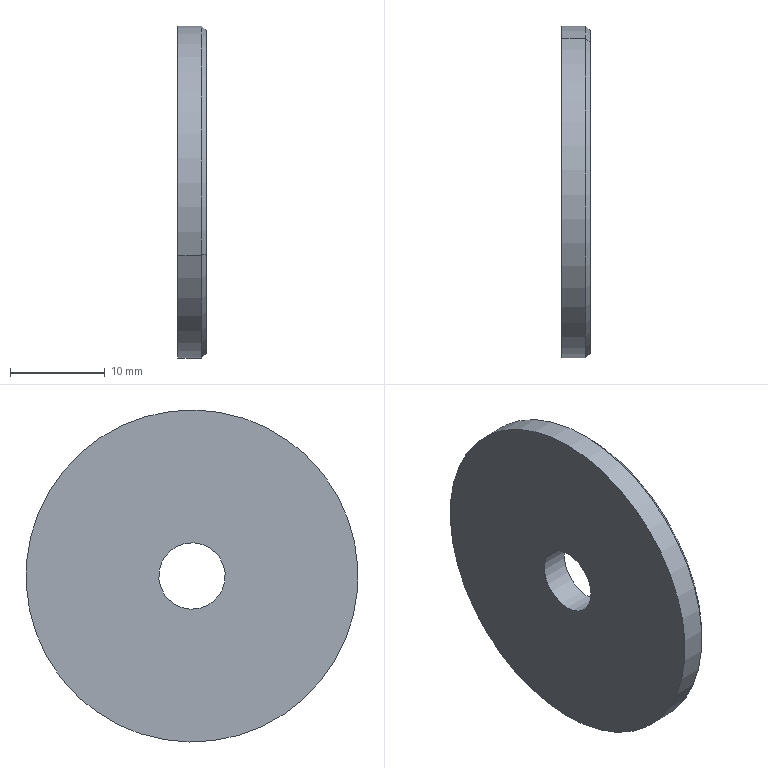Component | SolidWorks | DoubleFilmTransport-1_AxisEndCap-2 | 1 solid | 8 faces | box 3 x 35 x 35 mm | volume 2757 mm3 | cylinder 4 | cone 2 | plane 2 | commonest cylinder face diameters 35 x2 7 x2
build123d program:
from build123d import *


with BuildPart() as part:
    # Sketch1 → Revolve1 (revolve)
    with BuildSketch(Plane(origin=(0, 0, 0), x_dir=(1, 0, 0), z_dir=(0, 1, 0))):
        Polygon((3.5, -3), (17, -3), (17.5, -2.5), (17.5, 0), (3.5, 0), align=None)
    revolve(axis=Axis((0, 0, 0), (0, 0, 1)))


solid = part.part

# Placed as in the assembly
solid = solid.moved(Location((-468.246, 45.373, 13.5), (0, 90, 0)))
STEP:
#1=COLOUR_RGB('',0.7922,0.8196,0.9333);
#2=FILL_AREA_STYLE_COLOUR('',#1);
#3=FILL_AREA_STYLE('',(#2));
#4=SURFACE_STYLE_FILL_AREA(#3);
#5=SURFACE_SIDE_STYLE('',(#4));
#6=SURFACE_STYLE_USAGE(.BOTH.,#5);
#7=PRESENTATION_STYLE_ASSIGNMENT((#6));
#8=CARTESIAN_POINT('',(-18.435,1.15,0.2684));
#9=VERTEX_POINT('',#8);
#10=CARTESIAN_POINT('',(-18.435,2.423,0.7946));
#11=VERTEX_POINT('',#10);
#12=CARTESIAN_POINT('',(-18.435,1.786,0.5315));
#13=DIRECTION('',(1.,0.,0.));
#14=DIRECTION('',(0.,-0.9242,-0.3818));
#15=AXIS2_PLACEMENT_3D('',#12,#13,#14);
#16=CIRCLE('',#15,0.689);
#17=EDGE_CURVE('',#9,#11,#16,.T.);
#18=ORIENTED_EDGE('',*,*,#17,.T.);
#19=CARTESIAN_POINT('',(-18.336,2.423,0.7946));
#20=VERTEX_POINT('',#19);
#21=CARTESIAN_POINT('',(-18.435,2.423,0.7946));
#22=DIRECTION('',(1.,0.,0.));
#23=VECTOR('',#22,39.37);
#24=LINE('',#21,#23);
#25=EDGE_CURVE('',#11,#20,#24,.T.);
#26=ORIENTED_EDGE('',*,*,#25,.T.);
#27=CARTESIAN_POINT('',(-18.336,1.15,0.2684));
#28=VERTEX_POINT('',#27);
#29=CARTESIAN_POINT('',(-18.336,1.786,0.5315));
#30=DIRECTION('',(1.,0.,0.));
#31=DIRECTION('',(0.,-0.9242,-0.3818));
#32=AXIS2_PLACEMENT_3D('',#29,#30,#31);
#33=CIRCLE('',#32,0.689);
#34=EDGE_CURVE('',#28,#20,#33,.T.);
#35=ORIENTED_EDGE('',*,*,#34,.F.);
#36=CARTESIAN_POINT('',(-18.435,1.15,0.2684));
#37=DIRECTION('',(1.,0.,0.));
#38=VECTOR('',#37,39.37);
#39=LINE('',#36,#38);
#40=EDGE_CURVE('',#9,#28,#39,.T.);
#41=ORIENTED_EDGE('',*,*,#40,.F.);
#42=EDGE_LOOP('',(#18,#26,#35,#41));
#43=FACE_OUTER_BOUND('',#42,.T.);
#44=CARTESIAN_POINT('',(-18.435,1.786,0.5315));
#45=DIRECTION('',(1.,0.,0.));
#46=DIRECTION('',(0.,-0.9242,-0.3818));
#47=AXIS2_PLACEMENT_3D('',#44,#45,#46);
#48=CYLINDRICAL_SURFACE('',#47,0.689);
#49=ADVANCED_FACE('',(#43),#48,.T.);
#50=CARTESIAN_POINT('',(-18.317,1.168,0.2759));
#51=VERTEX_POINT('',#50);
#52=CARTESIAN_POINT('',(-18.317,2.405,0.7871));
#53=VERTEX_POINT('',#52);
#54=CARTESIAN_POINT('',(-18.317,1.786,0.5315));
#55=DIRECTION('',(1.,0.,0.));
#56=DIRECTION('',(0.,-0.9242,-0.3818));
#57=AXIS2_PLACEMENT_3D('',#54,#55,#56);
#58=CIRCLE('',#57,0.6693);
#59=EDGE_CURVE('',#51,#53,#58,.T.);
#60=ORIENTED_EDGE('',*,*,#59,.F.);
#61=CARTESIAN_POINT('',(-18.317,1.168,0.2759));
#62=DIRECTION('',(-0.7071,-0.6535,-0.27));
#63=VECTOR('',#62,39.37);
#64=LINE('',#61,#63);
#65=EDGE_CURVE('',#51,#28,#64,.T.);
#66=ORIENTED_EDGE('',*,*,#65,.T.);
#67=ORIENTED_EDGE('',*,*,#34,.T.);
#68=CARTESIAN_POINT('',(-18.317,2.405,0.7871));
#69=DIRECTION('',(-0.7071,0.6535,0.27));
#70=VECTOR('',#69,39.37);
#71=LINE('',#68,#70);
#72=EDGE_CURVE('',#53,#20,#71,.T.);
#73=ORIENTED_EDGE('',*,*,#72,.F.);
#74=EDGE_LOOP('',(#60,#66,#67,#73));
#75=FACE_OUTER_BOUND('',#74,.T.);
#76=CARTESIAN_POINT('',(-18.317,1.786,0.5315));
#77=DIRECTION('',(-1.,-0.,-0.));
#78=DIRECTION('',(0.,0.9242,0.3818));
#79=AXIS2_PLACEMENT_3D('',#76,#77,#78);
#80=CONICAL_SURFACE('',#79,0.6693,0.7854);
#81=ADVANCED_FACE('',(#75),#80,.T.);
#82=CARTESIAN_POINT('',(-18.435,1.914,0.5841));
#83=VERTEX_POINT('',#82);
#84=CARTESIAN_POINT('',(-18.435,1.659,0.4789));
#85=VERTEX_POINT('',#84);
#86=CARTESIAN_POINT('',(-18.435,1.786,0.5315));
#87=DIRECTION('',(1.,0.,0.));
#88=DIRECTION('',(0.,-0.9242,-0.3818));
#89=AXIS2_PLACEMENT_3D('',#86,#87,#88);
#90=CIRCLE('',#89,0.1378);
#91=EDGE_CURVE('',#83,#85,#90,.T.);
#92=ORIENTED_EDGE('',*,*,#91,.F.);
#93=CARTESIAN_POINT('',(-18.317,1.914,0.5841));
#94=VERTEX_POINT('',#93);
#95=CARTESIAN_POINT('',(-18.435,1.914,0.5841));
#96=DIRECTION('',(1.,0.,0.));
#97=VECTOR('',#96,39.37);
#98=LINE('',#95,#97);
#99=EDGE_CURVE('',#83,#94,#98,.T.);
#100=ORIENTED_EDGE('',*,*,#99,.T.);
#101=CARTESIAN_POINT('',(-18.317,1.659,0.4789));
#102=VERTEX_POINT('',#101);
#103=CARTESIAN_POINT('',(-18.317,1.786,0.5315));
#104=DIRECTION('',(1.,0.,0.));
#105=DIRECTION('',(0.,-0.9242,-0.3818));
#106=AXIS2_PLACEMENT_3D('',#103,#104,#105);
#107=CIRCLE('',#106,0.1378);
#108=EDGE_CURVE('',#94,#102,#107,.T.);
#109=ORIENTED_EDGE('',*,*,#108,.T.);
#110=CARTESIAN_POINT('',(-18.435,1.659,0.4789));
#111=DIRECTION('',(1.,0.,0.));
#112=VECTOR('',#111,39.37);
#113=LINE('',#110,#112);
#114=EDGE_CURVE('',#85,#102,#113,.T.);
#115=ORIENTED_EDGE('',*,*,#114,.F.);
#116=EDGE_LOOP('',(#92,#100,#109,#115));
#117=FACE_OUTER_BOUND('',#116,.T.);
#118=CARTESIAN_POINT('',(-18.435,1.786,0.5315));
#119=DIRECTION('',(1.,0.,0.));
#120=DIRECTION('',(0.,-0.9242,-0.3818));
#121=AXIS2_PLACEMENT_3D('',#118,#119,#120);
#122=CYLINDRICAL_SURFACE('',#121,0.1378);
#123=ADVANCED_FACE('',(#117),#122,.F.);
#124=ORIENTED_EDGE('',*,*,#99,.F.);
#125=CARTESIAN_POINT('',(-18.435,1.786,0.5315));
#126=DIRECTION('',(1.,0.,0.));
#127=DIRECTION('',(0.,-0.9242,-0.3818));
#128=AXIS2_PLACEMENT_3D('',#125,#126,#127);
#129=CIRCLE('',#128,0.1378);
#130=EDGE_CURVE('',#85,#83,#129,.T.);
#131=ORIENTED_EDGE('',*,*,#130,.F.);
#132=ORIENTED_EDGE('',*,*,#114,.T.);
#133=CARTESIAN_POINT('',(-18.317,1.786,0.5315));
#134=DIRECTION('',(1.,0.,0.));
#135=DIRECTION('',(0.,-0.9242,-0.3818));
#136=AXIS2_PLACEMENT_3D('',#133,#134,#135);
#137=CIRCLE('',#136,0.1378);
#138=EDGE_CURVE('',#102,#94,#137,.T.);
#139=ORIENTED_EDGE('',*,*,#138,.T.);
#140=EDGE_LOOP('',(#124,#131,#132,#139));
#141=FACE_OUTER_BOUND('',#140,.T.);
#142=CARTESIAN_POINT('',(-18.435,1.786,0.5315));
#143=DIRECTION('',(1.,0.,0.));
#144=DIRECTION('',(0.,-0.9242,-0.3818));
#145=AXIS2_PLACEMENT_3D('',#142,#143,#144);
#146=CYLINDRICAL_SURFACE('',#145,0.1378);
#147=ADVANCED_FACE('',(#141),#146,.F.);
#148=CARTESIAN_POINT('',(-18.317,1.786,0.5315));
#149=DIRECTION('',(1.,0.,0.));
#150=DIRECTION('',(0.,-0.9242,-0.3818));
#151=AXIS2_PLACEMENT_3D('',#148,#149,#150);
#152=CIRCLE('',#151,0.6693);
#153=EDGE_CURVE('',#53,#51,#152,.T.);
#154=ORIENTED_EDGE('',*,*,#153,.T.);
#155=ORIENTED_EDGE('',*,*,#59,.T.);
#156=EDGE_LOOP('',(#154,#155));
#157=FACE_OUTER_BOUND('',#156,.T.);
#158=ORIENTED_EDGE('',*,*,#138,.F.);
#159=ORIENTED_EDGE('',*,*,#108,.F.);
#160=EDGE_LOOP('',(#158,#159));
#161=FACE_BOUND('',#160,.T.);
#162=CARTESIAN_POINT('',(-18.317,1.659,0.4789));
#163=DIRECTION('',(1.,0.,0.));
#164=DIRECTION('',(0.,-0.9242,-0.3818));
#165=AXIS2_PLACEMENT_3D('',#162,#163,#164);
#166=PLANE('',#165);
#167=ADVANCED_FACE('',(#157,#161),#166,.T.);
#168=ORIENTED_EDGE('',*,*,#65,.F.);
#169=ORIENTED_EDGE('',*,*,#153,.F.);
#170=ORIENTED_EDGE('',*,*,#72,.T.);
#171=CARTESIAN_POINT('',(-18.336,1.786,0.5315));
#172=DIRECTION('',(1.,0.,0.));
#173=DIRECTION('',(0.,-0.9242,-0.3818));
#174=AXIS2_PLACEMENT_3D('',#171,#172,#173);
#175=CIRCLE('',#174,0.689);
#176=EDGE_CURVE('',#20,#28,#175,.T.);
#177=ORIENTED_EDGE('',*,*,#176,.T.);
#178=EDGE_LOOP('',(#168,#169,#170,#177));
#179=FACE_OUTER_BOUND('',#178,.T.);
#180=CARTESIAN_POINT('',(-18.317,1.786,0.5315));
#181=DIRECTION('',(-1.,-0.,-0.));
#182=DIRECTION('',(0.,0.9242,0.3818));
#183=AXIS2_PLACEMENT_3D('',#180,#181,#182);
#184=CONICAL_SURFACE('',#183,0.6693,0.7854);
#185=ADVANCED_FACE('',(#179),#184,.T.);
#186=ORIENTED_EDGE('',*,*,#25,.F.);
#187=CARTESIAN_POINT('',(-18.435,1.786,0.5315));
#188=DIRECTION('',(1.,0.,0.));
#189=DIRECTION('',(0.,-0.9242,-0.3818));
#190=AXIS2_PLACEMENT_3D('',#187,#188,#189);
#191=CIRCLE('',#190,0.689);
#192=EDGE_CURVE('',#11,#9,#191,.T.);
#193=ORIENTED_EDGE('',*,*,#192,.T.);
#194=ORIENTED_EDGE('',*,*,#40,.T.);
#195=ORIENTED_EDGE('',*,*,#176,.F.);
#196=EDGE_LOOP('',(#186,#193,#194,#195));
#197=FACE_OUTER_BOUND('',#196,.T.);
#198=CARTESIAN_POINT('',(-18.435,1.786,0.5315));
#199=DIRECTION('',(1.,0.,0.));
#200=DIRECTION('',(0.,-0.9242,-0.3818));
#201=AXIS2_PLACEMENT_3D('',#198,#199,#200);
#202=CYLINDRICAL_SURFACE('',#201,0.689);
#203=ADVANCED_FACE('',(#197),#202,.T.);
#204=ORIENTED_EDGE('',*,*,#130,.T.);
#205=ORIENTED_EDGE('',*,*,#91,.T.);
#206=EDGE_LOOP('',(#204,#205));
#207=FACE_BOUND('',#206,.T.);
#208=ORIENTED_EDGE('',*,*,#17,.F.);
#209=ORIENTED_EDGE('',*,*,#192,.F.);
#210=EDGE_LOOP('',(#208,#209));
#211=FACE_OUTER_BOUND('',#210,.T.);
#212=CARTESIAN_POINT('',(-18.435,1.15,0.2684));
#213=DIRECTION('',(-1.,-0.,-0.));
#214=DIRECTION('',(-0.,0.9242,0.3818));
#215=AXIS2_PLACEMENT_3D('',#212,#213,#214);
#216=PLANE('',#215);
#217=ADVANCED_FACE('',(#207,#211),#216,.T.);
#218=CLOSED_SHELL('',(#49,#81,#123,#147,#167,#185,#203,#217));
#219=MANIFOLD_SOLID_BREP('',#218);
#220=STYLED_ITEM('',(#7),#219);
#221=(LENGTH_UNIT()NAMED_UNIT(*)SI_UNIT($,.METRE.));
#222=LENGTH_MEASURE_WITH_UNIT(LENGTH_MEASURE(0.0254),#221);
#223=DIMENSIONAL_EXPONENTS(1.,0.,0.,0.,0.,0.,0.);
#224=(CONVERSION_BASED_UNIT('',#222)LENGTH_UNIT()NAMED_UNIT(#223));
#225=UNCERTAINTY_MEASURE_WITH_UNIT(LENGTH_MEASURE(0.00001),#224,'','');
#226=(NAMED_UNIT(*)PLANE_ANGLE_UNIT()SI_UNIT($,.RADIAN.));
#227=(NAMED_UNIT(*)SI_UNIT($,.STERADIAN.)SOLID_ANGLE_UNIT());
#228=(GEOMETRIC_REPRESENTATION_CONTEXT(3)GLOBAL_UNCERTAINTY_ASSIGNED_CONTEXT((#225))GLOBAL_UNIT_ASSIGNED_CONTEXT((#224,#226,#227))REPRESENTATION_CONTEXT('',''));
#229=MECHANICAL_DESIGN_GEOMETRIC_PRESENTATION_REPRESENTATION('',(#220),#228);
#230=CARTESIAN_POINT('',(0.,0.,0.));
#231=DIRECTION('',(0.,0.,1.));
#232=DIRECTION('',(1.,0.,0.));
#233=AXIS2_PLACEMENT_3D('',#230,#231,#232);
#234=(LENGTH_UNIT()NAMED_UNIT(*)SI_UNIT($,.METRE.));
#235=LENGTH_MEASURE_WITH_UNIT(LENGTH_MEASURE(0.0254),#234);
#236=DIMENSIONAL_EXPONENTS(1.,0.,0.,0.,0.,0.,0.);
#237=(CONVERSION_BASED_UNIT('',#235)LENGTH_UNIT()NAMED_UNIT(#236));
#238=UNCERTAINTY_MEASURE_WITH_UNIT(LENGTH_MEASURE(0.00001),#237,'','');
#239=(NAMED_UNIT(*)PLANE_ANGLE_UNIT()SI_UNIT($,.RADIAN.));
#240=(NAMED_UNIT(*)SI_UNIT($,.STERADIAN.)SOLID_ANGLE_UNIT());
#241=(GEOMETRIC_REPRESENTATION_CONTEXT(3)GLOBAL_UNCERTAINTY_ASSIGNED_CONTEXT((#238))GLOBAL_UNIT_ASSIGNED_CONTEXT((#237,#239,#240))REPRESENTATION_CONTEXT('',''));
#242=ADVANCED_BREP_SHAPE_REPRESENTATION('',(#219,#233),#241);
#243=PRESENTATION_LAYER_ASSIGNMENT('','',(#220));